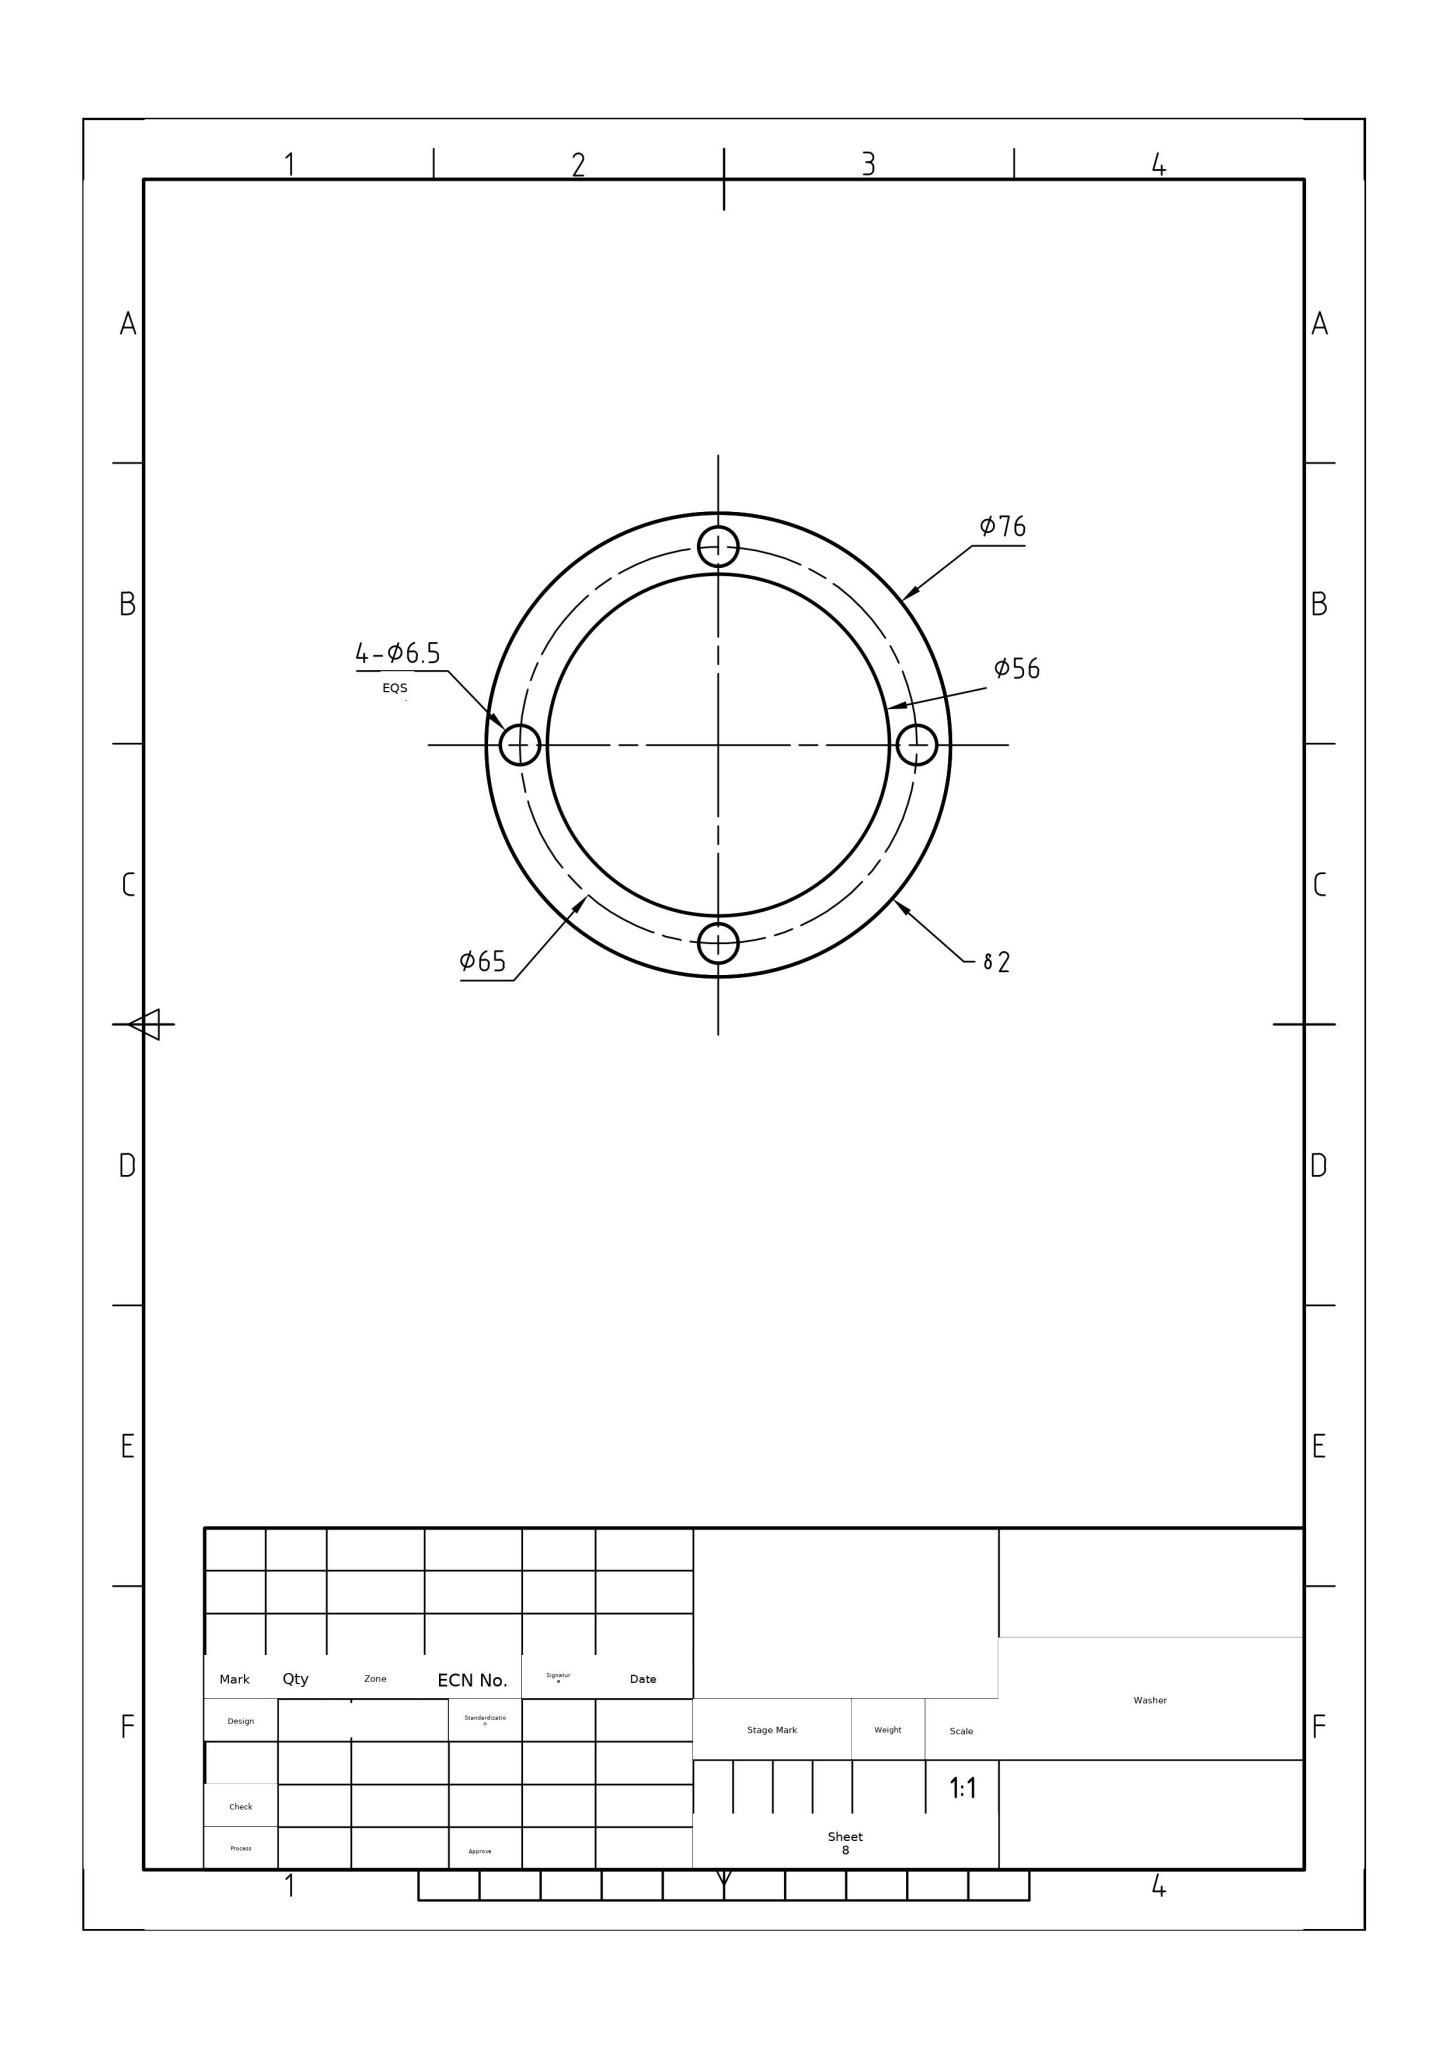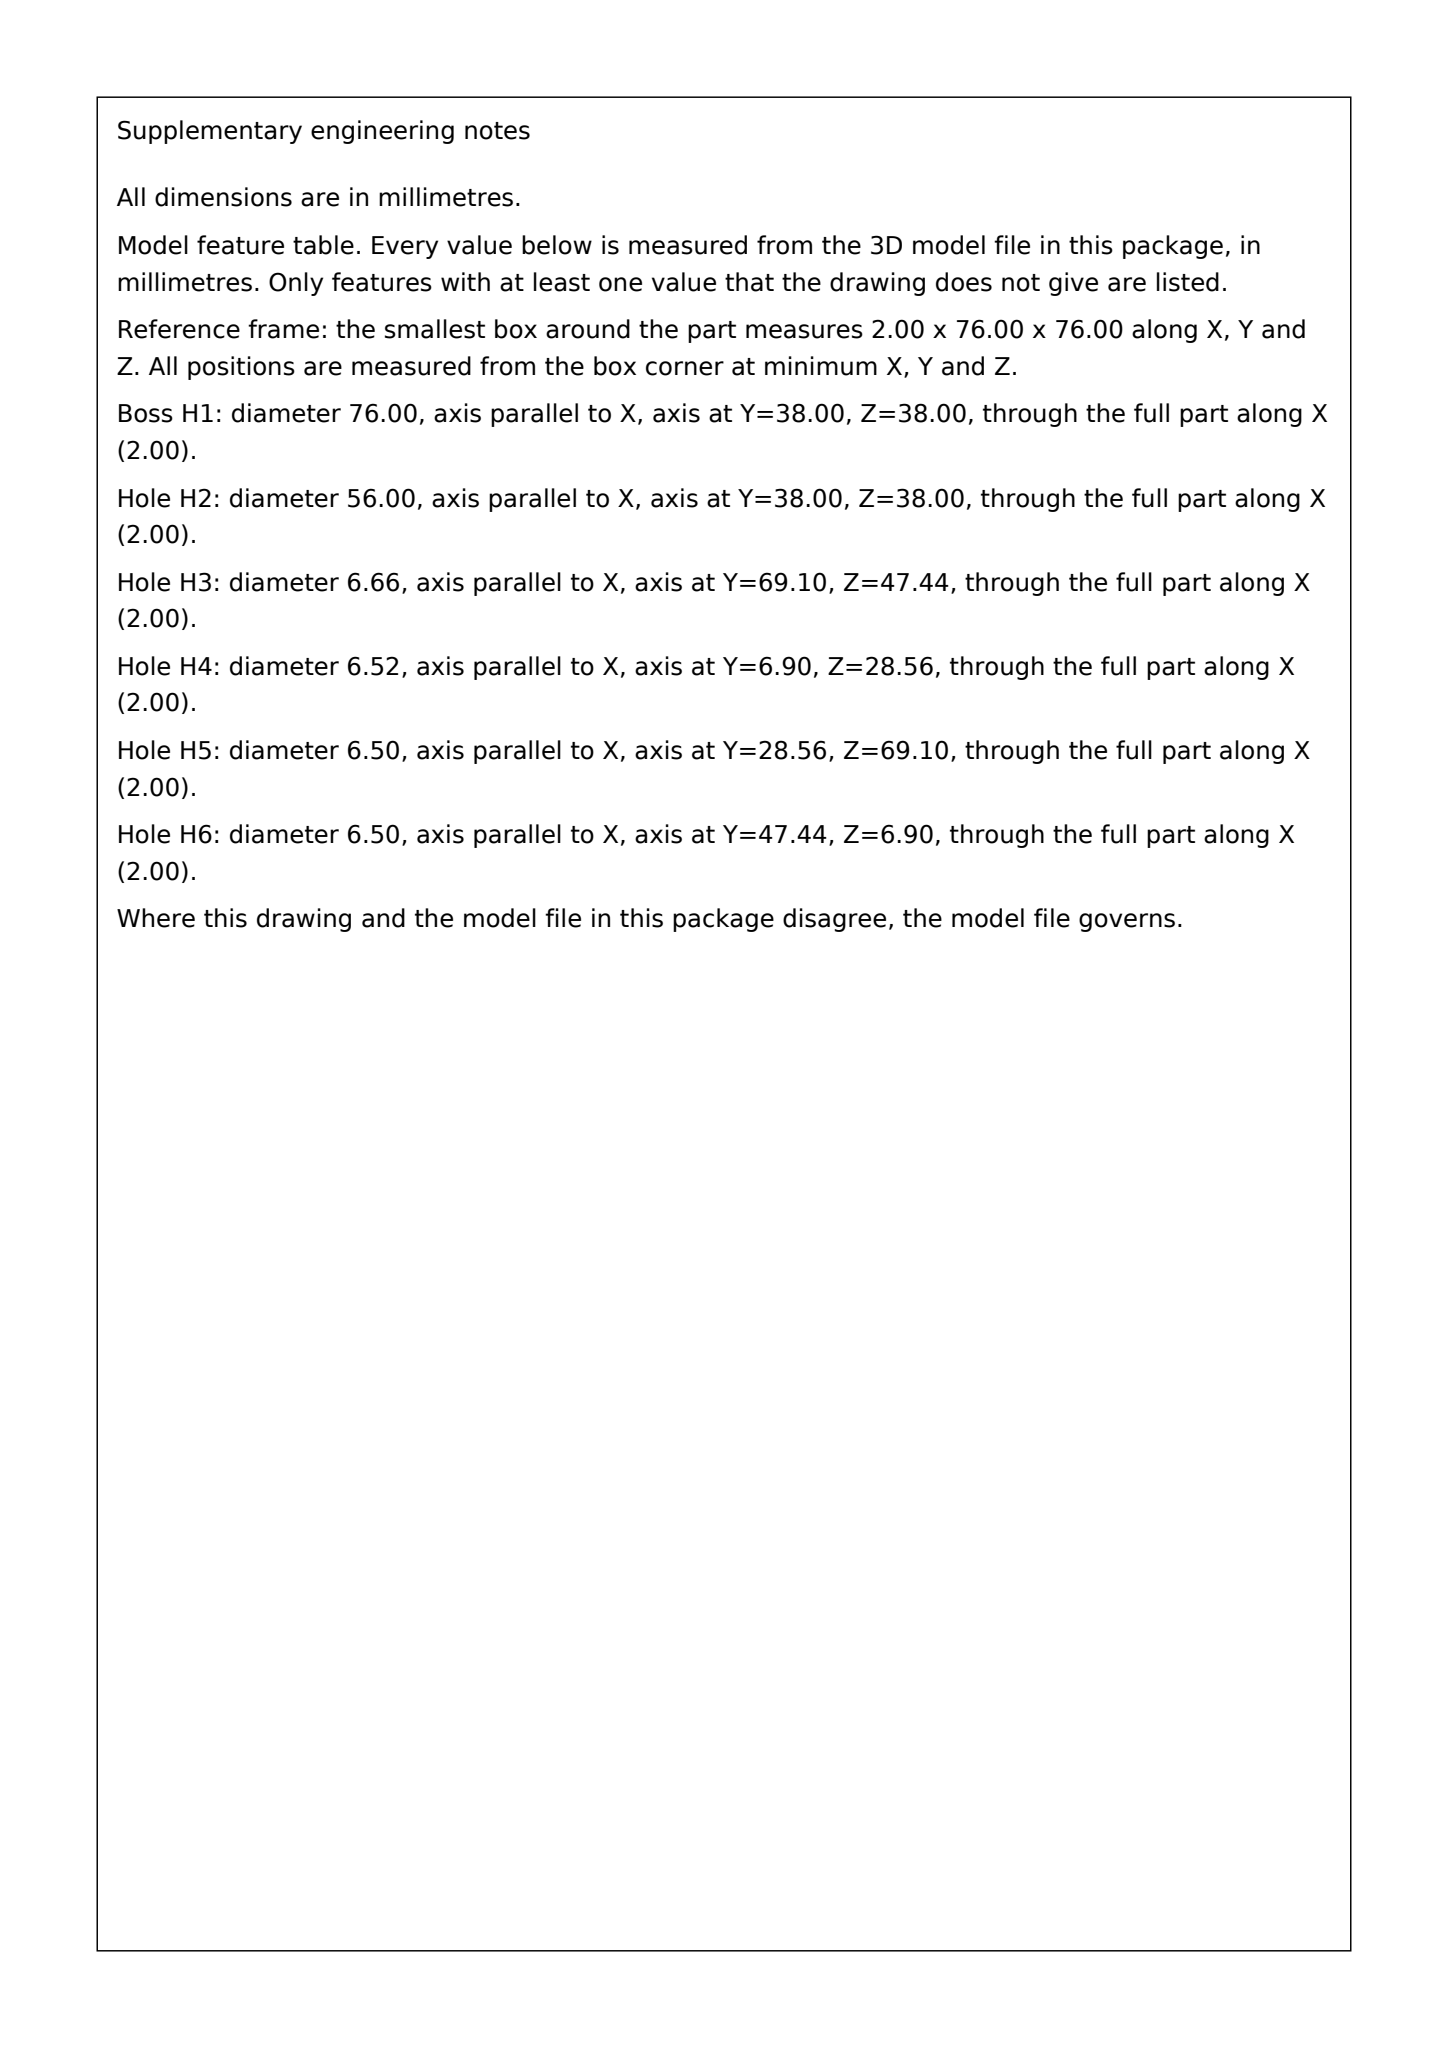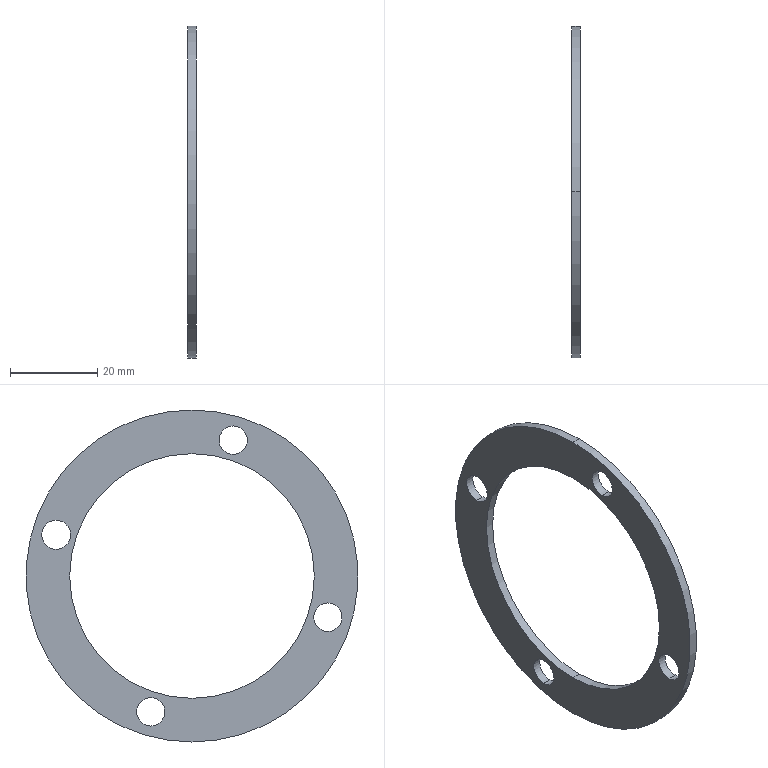Part | SolidWorks | mm | 1 solid | 14 faces | box 2 x 76 x 76 mm | volume 3878 mm3 | cylinder 12 | plane 2 | commonest cylinder face diameters 6.5 x4 6.651 x2 6.516 x2 56 x2 76 x2
build123d program:
from build123d import *

# Parameters (mm, degrees)
SKETCH2_R           = 38
SKETCH2_R_2         = 28
BOSS_EXTRUDE1_DEPTH = 2
CUT_EXTRUDE1_REACH  = 55.777
SKETCH3_R           = 3.326
SKETCH3_R_2         = 3.25
SKETCH3_R_3         = 3.258


with BuildPart() as part:
    # Sketch2 → Boss-Extrude1 (new body)
    with BuildSketch(Plane(origin=(0, 0, 0), x_dir=(0, 0, -1), z_dir=(1, 0, 0))):
        Circle(SKETCH2_R)
        Circle(SKETCH2_R_2, mode=Mode.SUBTRACT)
    extrude(amount=BOSS_EXTRUDE1_DEPTH)

    # Sketch3 → Cut-Extrude1 (cut, up to next)
    with BuildSketch(Plane.ZY, mode=Mode.PRIVATE) as cut_extrude1_sk1:
        with Locations((9.437, 31.1)):
            Circle(SKETCH3_R)
    cut_extrude1_tool1 = extrude(cut_extrude1_sk1.sketch, amount=-CUT_EXTRUDE1_REACH, mode=Mode.PRIVATE) & part.part
    # Sketch3 → Cut-Extrude1 (cut, up to next)
    with BuildSketch(Plane.ZY, mode=Mode.PRIVATE) as cut_extrude1_sk2:
        with Locations((31.1, -9.437)):
            Circle(SKETCH3_R_2)
    cut_extrude1_tool2 = extrude(cut_extrude1_sk2.sketch, amount=-CUT_EXTRUDE1_REACH, mode=Mode.PRIVATE) & part.part
    # Sketch3 → Cut-Extrude1 (cut, up to next)
    with BuildSketch(Plane.ZY, mode=Mode.PRIVATE) as cut_extrude1_sk3:
        with Locations((-9.437, -31.1)):
            Circle(SKETCH3_R_3)
    cut_extrude1_tool3 = extrude(cut_extrude1_sk3.sketch, amount=-CUT_EXTRUDE1_REACH, mode=Mode.PRIVATE) & part.part
    # Sketch3 → Cut-Extrude1 (cut, up to next)
    with BuildSketch(Plane.ZY, mode=Mode.PRIVATE) as cut_extrude1_sk4:
        with Locations((-31.1, 9.437)):
            Circle(SKETCH3_R_2)
    cut_extrude1_tool4 = extrude(cut_extrude1_sk4.sketch, amount=-CUT_EXTRUDE1_REACH, mode=Mode.PRIVATE) & part.part
    add(cut_extrude1_tool1.solids().sort_by_distance((0, 31.1, 9.437))[0], mode=Mode.SUBTRACT)
    add(cut_extrude1_tool2.solids().sort_by_distance((0, -9.437, 31.1))[0], mode=Mode.SUBTRACT)
    add(cut_extrude1_tool3.solids().sort_by_distance((0, -31.1, -9.437))[0], mode=Mode.SUBTRACT)
    add(cut_extrude1_tool4.solids().sort_by_distance((0, 9.437, -31.1))[0], mode=Mode.SUBTRACT)


solid = part.part
STEP:
#1=CARTESIAN_POINT('',(2.,31.1,6.111));
#2=VERTEX_POINT('',#1);
#3=CARTESIAN_POINT('',(2.,31.1,12.763));
#4=VERTEX_POINT('',#3);
#5=CARTESIAN_POINT('',(2.,31.1,9.437));
#6=DIRECTION('',(-1.,0.,0.));
#7=DIRECTION('',(0.,0.,-1.));
#8=AXIS2_PLACEMENT_3D('',#5,#6,#7);
#9=CIRCLE('',#8,3.326);
#10=EDGE_CURVE('',#2,#4,#9,.T.);
#11=ORIENTED_EDGE('',*,*,#10,.F.);
#12=CARTESIAN_POINT('',(0.,31.1,6.111));
#13=VERTEX_POINT('',#12);
#14=CARTESIAN_POINT('',(2.001,31.1,6.111));
#15=DIRECTION('',(-1.,0.,0.));
#16=VECTOR('',#15,1000.);
#17=LINE('',#14,#16);
#18=EDGE_CURVE('',#2,#13,#17,.T.);
#19=ORIENTED_EDGE('',*,*,#18,.T.);
#20=CARTESIAN_POINT('',(0.,31.1,12.763));
#21=VERTEX_POINT('',#20);
#22=CARTESIAN_POINT('',(0.,31.1,9.437));
#23=DIRECTION('',(-1.,0.,0.));
#24=DIRECTION('',(0.,0.,1.));
#25=AXIS2_PLACEMENT_3D('',#22,#23,#24);
#26=CIRCLE('',#25,3.326);
#27=EDGE_CURVE('',#13,#21,#26,.T.);
#28=ORIENTED_EDGE('',*,*,#27,.T.);
#29=CARTESIAN_POINT('',(2.001,31.1,12.763));
#30=DIRECTION('',(-1.,0.,0.));
#31=VECTOR('',#30,1000.);
#32=LINE('',#29,#31);
#33=EDGE_CURVE('',#4,#21,#32,.T.);
#34=ORIENTED_EDGE('',*,*,#33,.F.);
#35=EDGE_LOOP('',(#11,#19,#28,#34));
#36=FACE_OUTER_BOUND('',#35,.T.);
#37=CARTESIAN_POINT('',(2.001,31.1,9.437));
#38=DIRECTION('',(-1.,0.,0.));
#39=DIRECTION('',(0.,0.,1.));
#40=AXIS2_PLACEMENT_3D('',#37,#38,#39);
#41=CYLINDRICAL_SURFACE('',#40,3.326);
#42=ADVANCED_FACE('',(#36),#41,.F.);
#43=CARTESIAN_POINT('',(2.,-9.437,27.85));
#44=VERTEX_POINT('',#43);
#45=CARTESIAN_POINT('',(2.,-9.437,34.35));
#46=VERTEX_POINT('',#45);
#47=CARTESIAN_POINT('',(2.,-9.437,31.1));
#48=DIRECTION('',(-1.,0.,0.));
#49=DIRECTION('',(0.,0.,-1.));
#50=AXIS2_PLACEMENT_3D('',#47,#48,#49);
#51=CIRCLE('',#50,3.25);
#52=EDGE_CURVE('',#44,#46,#51,.T.);
#53=ORIENTED_EDGE('',*,*,#52,.F.);
#54=CARTESIAN_POINT('',(0.,-9.437,27.85));
#55=VERTEX_POINT('',#54);
#56=CARTESIAN_POINT('',(2.001,-9.437,27.85));
#57=DIRECTION('',(-1.,0.,0.));
#58=VECTOR('',#57,1000.);
#59=LINE('',#56,#58);
#60=EDGE_CURVE('',#44,#55,#59,.T.);
#61=ORIENTED_EDGE('',*,*,#60,.T.);
#62=CARTESIAN_POINT('',(0.,-9.437,34.35));
#63=VERTEX_POINT('',#62);
#64=CARTESIAN_POINT('',(0.,-9.437,31.1));
#65=DIRECTION('',(-1.,0.,0.));
#66=DIRECTION('',(0.,0.,1.));
#67=AXIS2_PLACEMENT_3D('',#64,#65,#66);
#68=CIRCLE('',#67,3.25);
#69=EDGE_CURVE('',#55,#63,#68,.T.);
#70=ORIENTED_EDGE('',*,*,#69,.T.);
#71=CARTESIAN_POINT('',(2.001,-9.437,34.35));
#72=DIRECTION('',(-1.,0.,0.));
#73=VECTOR('',#72,1000.);
#74=LINE('',#71,#73);
#75=EDGE_CURVE('',#46,#63,#74,.T.);
#76=ORIENTED_EDGE('',*,*,#75,.F.);
#77=EDGE_LOOP('',(#53,#61,#70,#76));
#78=FACE_OUTER_BOUND('',#77,.T.);
#79=CARTESIAN_POINT('',(2.001,-9.437,31.1));
#80=DIRECTION('',(-1.,0.,0.));
#81=DIRECTION('',(0.,0.,1.));
#82=AXIS2_PLACEMENT_3D('',#79,#80,#81);
#83=CYLINDRICAL_SURFACE('',#82,3.25);
#84=ADVANCED_FACE('',(#78),#83,.F.);
#85=CARTESIAN_POINT('',(2.,-31.1,-12.695));
#86=VERTEX_POINT('',#85);
#87=CARTESIAN_POINT('',(2.,-31.1,-6.179));
#88=VERTEX_POINT('',#87);
#89=CARTESIAN_POINT('',(2.,-31.1,-9.437));
#90=DIRECTION('',(-1.,0.,0.));
#91=DIRECTION('',(0.,0.,-1.));
#92=AXIS2_PLACEMENT_3D('',#89,#90,#91);
#93=CIRCLE('',#92,3.258);
#94=EDGE_CURVE('',#86,#88,#93,.T.);
#95=ORIENTED_EDGE('',*,*,#94,.F.);
#96=CARTESIAN_POINT('',(0.,-31.1,-12.695));
#97=VERTEX_POINT('',#96);
#98=CARTESIAN_POINT('',(2.001,-31.1,-12.695));
#99=DIRECTION('',(-1.,0.,0.));
#100=VECTOR('',#99,1000.);
#101=LINE('',#98,#100);
#102=EDGE_CURVE('',#86,#97,#101,.T.);
#103=ORIENTED_EDGE('',*,*,#102,.T.);
#104=CARTESIAN_POINT('',(0.,-31.1,-6.179));
#105=VERTEX_POINT('',#104);
#106=CARTESIAN_POINT('',(0.,-31.1,-9.437));
#107=DIRECTION('',(-1.,0.,0.));
#108=DIRECTION('',(0.,0.,1.));
#109=AXIS2_PLACEMENT_3D('',#106,#107,#108);
#110=CIRCLE('',#109,3.258);
#111=EDGE_CURVE('',#97,#105,#110,.T.);
#112=ORIENTED_EDGE('',*,*,#111,.T.);
#113=CARTESIAN_POINT('',(2.001,-31.1,-6.179));
#114=DIRECTION('',(-1.,0.,0.));
#115=VECTOR('',#114,1000.);
#116=LINE('',#113,#115);
#117=EDGE_CURVE('',#88,#105,#116,.T.);
#118=ORIENTED_EDGE('',*,*,#117,.F.);
#119=EDGE_LOOP('',(#95,#103,#112,#118));
#120=FACE_OUTER_BOUND('',#119,.T.);
#121=CARTESIAN_POINT('',(2.001,-31.1,-9.437));
#122=DIRECTION('',(-1.,0.,0.));
#123=DIRECTION('',(0.,0.,1.));
#124=AXIS2_PLACEMENT_3D('',#121,#122,#123);
#125=CYLINDRICAL_SURFACE('',#124,3.258);
#126=ADVANCED_FACE('',(#120),#125,.F.);
#127=CARTESIAN_POINT('',(2.,9.437,-34.35));
#128=VERTEX_POINT('',#127);
#129=CARTESIAN_POINT('',(2.,9.437,-27.85));
#130=VERTEX_POINT('',#129);
#131=CARTESIAN_POINT('',(2.,9.437,-31.1));
#132=DIRECTION('',(-1.,0.,0.));
#133=DIRECTION('',(0.,0.,-1.));
#134=AXIS2_PLACEMENT_3D('',#131,#132,#133);
#135=CIRCLE('',#134,3.25);
#136=EDGE_CURVE('',#128,#130,#135,.T.);
#137=ORIENTED_EDGE('',*,*,#136,.F.);
#138=CARTESIAN_POINT('',(0.,9.437,-34.35));
#139=VERTEX_POINT('',#138);
#140=CARTESIAN_POINT('',(2.001,9.437,-34.35));
#141=DIRECTION('',(-1.,0.,0.));
#142=VECTOR('',#141,1000.);
#143=LINE('',#140,#142);
#144=EDGE_CURVE('',#128,#139,#143,.T.);
#145=ORIENTED_EDGE('',*,*,#144,.T.);
#146=CARTESIAN_POINT('',(0.,9.437,-27.85));
#147=VERTEX_POINT('',#146);
#148=CARTESIAN_POINT('',(0.,9.437,-31.1));
#149=DIRECTION('',(-1.,0.,0.));
#150=DIRECTION('',(0.,0.,1.));
#151=AXIS2_PLACEMENT_3D('',#148,#149,#150);
#152=CIRCLE('',#151,3.25);
#153=EDGE_CURVE('',#139,#147,#152,.T.);
#154=ORIENTED_EDGE('',*,*,#153,.T.);
#155=CARTESIAN_POINT('',(2.001,9.437,-27.85));
#156=DIRECTION('',(-1.,0.,0.));
#157=VECTOR('',#156,1000.);
#158=LINE('',#155,#157);
#159=EDGE_CURVE('',#130,#147,#158,.T.);
#160=ORIENTED_EDGE('',*,*,#159,.F.);
#161=EDGE_LOOP('',(#137,#145,#154,#160));
#162=FACE_OUTER_BOUND('',#161,.T.);
#163=CARTESIAN_POINT('',(2.001,9.437,-31.1));
#164=DIRECTION('',(-1.,0.,0.));
#165=DIRECTION('',(0.,0.,1.));
#166=AXIS2_PLACEMENT_3D('',#163,#164,#165);
#167=CYLINDRICAL_SURFACE('',#166,3.25);
#168=ADVANCED_FACE('',(#162),#167,.F.);
#169=CARTESIAN_POINT('',(2.,0.,28.));
#170=VERTEX_POINT('',#169);
#171=CARTESIAN_POINT('',(2.,0.,-28.));
#172=VERTEX_POINT('',#171);
#173=CARTESIAN_POINT('',(2.,0.,0.));
#174=DIRECTION('',(1.,0.,0.));
#175=DIRECTION('',(0.,0.,-1.));
#176=AXIS2_PLACEMENT_3D('',#173,#174,#175);
#177=CIRCLE('',#176,28.);
#178=EDGE_CURVE('',#170,#172,#177,.T.);
#179=ORIENTED_EDGE('',*,*,#178,.T.);
#180=CARTESIAN_POINT('',(0.,0.,-28.));
#181=VERTEX_POINT('',#180);
#182=CARTESIAN_POINT('',(2.,0.,-28.));
#183=DIRECTION('',(-1.,0.,0.));
#184=VECTOR('',#183,1000.);
#185=LINE('',#182,#184);
#186=EDGE_CURVE('',#172,#181,#185,.T.);
#187=ORIENTED_EDGE('',*,*,#186,.T.);
#188=CARTESIAN_POINT('',(0.,0.,28.));
#189=VERTEX_POINT('',#188);
#190=CARTESIAN_POINT('',(0.,0.,0.));
#191=DIRECTION('',(1.,0.,0.));
#192=DIRECTION('',(0.,0.,-1.));
#193=AXIS2_PLACEMENT_3D('',#190,#191,#192);
#194=CIRCLE('',#193,28.);
#195=EDGE_CURVE('',#189,#181,#194,.T.);
#196=ORIENTED_EDGE('',*,*,#195,.F.);
#197=CARTESIAN_POINT('',(2.,0.,28.));
#198=DIRECTION('',(-1.,0.,0.));
#199=VECTOR('',#198,1000.);
#200=LINE('',#197,#199);
#201=EDGE_CURVE('',#170,#189,#200,.T.);
#202=ORIENTED_EDGE('',*,*,#201,.F.);
#203=EDGE_LOOP('',(#179,#187,#196,#202));
#204=FACE_OUTER_BOUND('',#203,.T.);
#205=CARTESIAN_POINT('',(2.,0.,0.));
#206=DIRECTION('',(-1.,0.,0.));
#207=DIRECTION('',(0.,0.,1.));
#208=AXIS2_PLACEMENT_3D('',#205,#206,#207);
#209=CYLINDRICAL_SURFACE('',#208,28.);
#210=ADVANCED_FACE('',(#204),#209,.F.);
#211=CARTESIAN_POINT('',(2.,0.,-38.));
#212=VERTEX_POINT('',#211);
#213=CARTESIAN_POINT('',(2.,0.,38.));
#214=VERTEX_POINT('',#213);
#215=CARTESIAN_POINT('',(2.,0.,0.));
#216=DIRECTION('',(1.,0.,0.));
#217=DIRECTION('',(0.,0.,-1.));
#218=AXIS2_PLACEMENT_3D('',#215,#216,#217);
#219=CIRCLE('',#218,38.);
#220=EDGE_CURVE('',#212,#214,#219,.T.);
#221=ORIENTED_EDGE('',*,*,#220,.F.);
#222=CARTESIAN_POINT('',(0.,0.,-38.));
#223=VERTEX_POINT('',#222);
#224=CARTESIAN_POINT('',(2.,0.,-38.));
#225=DIRECTION('',(-1.,0.,0.));
#226=VECTOR('',#225,1000.);
#227=LINE('',#224,#226);
#228=EDGE_CURVE('',#212,#223,#227,.T.);
#229=ORIENTED_EDGE('',*,*,#228,.T.);
#230=CARTESIAN_POINT('',(0.,0.,38.));
#231=VERTEX_POINT('',#230);
#232=CARTESIAN_POINT('',(0.,0.,0.));
#233=DIRECTION('',(1.,0.,0.));
#234=DIRECTION('',(0.,0.,-1.));
#235=AXIS2_PLACEMENT_3D('',#232,#233,#234);
#236=CIRCLE('',#235,38.);
#237=EDGE_CURVE('',#223,#231,#236,.T.);
#238=ORIENTED_EDGE('',*,*,#237,.T.);
#239=CARTESIAN_POINT('',(2.,0.,38.));
#240=DIRECTION('',(-1.,0.,0.));
#241=VECTOR('',#240,1000.);
#242=LINE('',#239,#241);
#243=EDGE_CURVE('',#214,#231,#242,.T.);
#244=ORIENTED_EDGE('',*,*,#243,.F.);
#245=EDGE_LOOP('',(#221,#229,#238,#244));
#246=FACE_OUTER_BOUND('',#245,.T.);
#247=CARTESIAN_POINT('',(2.,0.,0.));
#248=DIRECTION('',(-1.,0.,0.));
#249=DIRECTION('',(0.,0.,1.));
#250=AXIS2_PLACEMENT_3D('',#247,#248,#249);
#251=CYLINDRICAL_SURFACE('',#250,38.);
#252=ADVANCED_FACE('',(#246),#251,.T.);
#253=CARTESIAN_POINT('',(2.,31.1,9.437));
#254=DIRECTION('',(-1.,0.,0.));
#255=DIRECTION('',(0.,0.,-1.));
#256=AXIS2_PLACEMENT_3D('',#253,#254,#255);
#257=CIRCLE('',#256,3.326);
#258=EDGE_CURVE('',#4,#2,#257,.T.);
#259=ORIENTED_EDGE('',*,*,#258,.T.);
#260=ORIENTED_EDGE('',*,*,#10,.T.);
#261=EDGE_LOOP('',(#259,#260));
#262=FACE_BOUND('',#261,.T.);
#263=CARTESIAN_POINT('',(2.,-9.437,31.1));
#264=DIRECTION('',(-1.,0.,0.));
#265=DIRECTION('',(0.,0.,-1.));
#266=AXIS2_PLACEMENT_3D('',#263,#264,#265);
#267=CIRCLE('',#266,3.25);
#268=EDGE_CURVE('',#46,#44,#267,.T.);
#269=ORIENTED_EDGE('',*,*,#268,.T.);
#270=ORIENTED_EDGE('',*,*,#52,.T.);
#271=EDGE_LOOP('',(#269,#270));
#272=FACE_BOUND('',#271,.T.);
#273=CARTESIAN_POINT('',(2.,-31.1,-9.437));
#274=DIRECTION('',(-1.,0.,0.));
#275=DIRECTION('',(0.,0.,-1.));
#276=AXIS2_PLACEMENT_3D('',#273,#274,#275);
#277=CIRCLE('',#276,3.258);
#278=EDGE_CURVE('',#88,#86,#277,.T.);
#279=ORIENTED_EDGE('',*,*,#278,.T.);
#280=ORIENTED_EDGE('',*,*,#94,.T.);
#281=EDGE_LOOP('',(#279,#280));
#282=FACE_BOUND('',#281,.T.);
#283=CARTESIAN_POINT('',(2.,9.437,-31.1));
#284=DIRECTION('',(-1.,0.,0.));
#285=DIRECTION('',(0.,0.,-1.));
#286=AXIS2_PLACEMENT_3D('',#283,#284,#285);
#287=CIRCLE('',#286,3.25);
#288=EDGE_CURVE('',#130,#128,#287,.T.);
#289=ORIENTED_EDGE('',*,*,#288,.T.);
#290=ORIENTED_EDGE('',*,*,#136,.T.);
#291=EDGE_LOOP('',(#289,#290));
#292=FACE_BOUND('',#291,.T.);
#293=CARTESIAN_POINT('',(2.,0.,0.));
#294=DIRECTION('',(1.,0.,0.));
#295=DIRECTION('',(0.,0.,-1.));
#296=AXIS2_PLACEMENT_3D('',#293,#294,#295);
#297=CIRCLE('',#296,38.);
#298=EDGE_CURVE('',#214,#212,#297,.T.);
#299=ORIENTED_EDGE('',*,*,#298,.T.);
#300=ORIENTED_EDGE('',*,*,#220,.T.);
#301=EDGE_LOOP('',(#299,#300));
#302=FACE_OUTER_BOUND('',#301,.T.);
#303=ORIENTED_EDGE('',*,*,#178,.F.);
#304=CARTESIAN_POINT('',(2.,0.,0.));
#305=DIRECTION('',(1.,0.,0.));
#306=DIRECTION('',(0.,0.,-1.));
#307=AXIS2_PLACEMENT_3D('',#304,#305,#306);
#308=CIRCLE('',#307,28.);
#309=EDGE_CURVE('',#172,#170,#308,.T.);
#310=ORIENTED_EDGE('',*,*,#309,.F.);
#311=EDGE_LOOP('',(#303,#310));
#312=FACE_BOUND('',#311,.T.);
#313=CARTESIAN_POINT('',(2.,0.,0.));
#314=DIRECTION('',(1.,0.,0.));
#315=DIRECTION('',(0.,0.,-1.));
#316=AXIS2_PLACEMENT_3D('',#313,#314,#315);
#317=PLANE('',#316);
#318=ADVANCED_FACE('',(#262,#272,#282,#292,#302,#312),#317,.T.);
#319=CARTESIAN_POINT('',(0.,31.1,9.437));
#320=DIRECTION('',(-1.,0.,0.));
#321=DIRECTION('',(0.,0.,1.));
#322=AXIS2_PLACEMENT_3D('',#319,#320,#321);
#323=CIRCLE('',#322,3.326);
#324=EDGE_CURVE('',#21,#13,#323,.T.);
#325=ORIENTED_EDGE('',*,*,#324,.F.);
#326=ORIENTED_EDGE('',*,*,#27,.F.);
#327=EDGE_LOOP('',(#325,#326));
#328=FACE_BOUND('',#327,.T.);
#329=CARTESIAN_POINT('',(0.,-9.437,31.1));
#330=DIRECTION('',(-1.,0.,0.));
#331=DIRECTION('',(0.,0.,1.));
#332=AXIS2_PLACEMENT_3D('',#329,#330,#331);
#333=CIRCLE('',#332,3.25);
#334=EDGE_CURVE('',#63,#55,#333,.T.);
#335=ORIENTED_EDGE('',*,*,#334,.F.);
#336=ORIENTED_EDGE('',*,*,#69,.F.);
#337=EDGE_LOOP('',(#335,#336));
#338=FACE_BOUND('',#337,.T.);
#339=CARTESIAN_POINT('',(0.,-31.1,-9.437));
#340=DIRECTION('',(-1.,0.,0.));
#341=DIRECTION('',(0.,0.,1.));
#342=AXIS2_PLACEMENT_3D('',#339,#340,#341);
#343=CIRCLE('',#342,3.258);
#344=EDGE_CURVE('',#105,#97,#343,.T.);
#345=ORIENTED_EDGE('',*,*,#344,.F.);
#346=ORIENTED_EDGE('',*,*,#111,.F.);
#347=EDGE_LOOP('',(#345,#346));
#348=FACE_BOUND('',#347,.T.);
#349=CARTESIAN_POINT('',(0.,9.437,-31.1));
#350=DIRECTION('',(-1.,0.,0.));
#351=DIRECTION('',(0.,0.,1.));
#352=AXIS2_PLACEMENT_3D('',#349,#350,#351);
#353=CIRCLE('',#352,3.25);
#354=EDGE_CURVE('',#147,#139,#353,.T.);
#355=ORIENTED_EDGE('',*,*,#354,.F.);
#356=ORIENTED_EDGE('',*,*,#153,.F.);
#357=EDGE_LOOP('',(#355,#356));
#358=FACE_BOUND('',#357,.T.);
#359=CARTESIAN_POINT('',(0.,0.,0.));
#360=DIRECTION('',(1.,0.,0.));
#361=DIRECTION('',(0.,0.,-1.));
#362=AXIS2_PLACEMENT_3D('',#359,#360,#361);
#363=CIRCLE('',#362,38.);
#364=EDGE_CURVE('',#231,#223,#363,.T.);
#365=ORIENTED_EDGE('',*,*,#364,.F.);
#366=ORIENTED_EDGE('',*,*,#237,.F.);
#367=EDGE_LOOP('',(#365,#366));
#368=FACE_OUTER_BOUND('',#367,.T.);
#369=ORIENTED_EDGE('',*,*,#195,.T.);
#370=CARTESIAN_POINT('',(0.,0.,0.));
#371=DIRECTION('',(1.,0.,0.));
#372=DIRECTION('',(0.,0.,-1.));
#373=AXIS2_PLACEMENT_3D('',#370,#371,#372);
#374=CIRCLE('',#373,28.);
#375=EDGE_CURVE('',#181,#189,#374,.T.);
#376=ORIENTED_EDGE('',*,*,#375,.T.);
#377=EDGE_LOOP('',(#369,#376));
#378=FACE_BOUND('',#377,.T.);
#379=CARTESIAN_POINT('',(0.,0.,0.));
#380=DIRECTION('',(1.,0.,0.));
#381=DIRECTION('',(0.,0.,-1.));
#382=AXIS2_PLACEMENT_3D('',#379,#380,#381);
#383=PLANE('',#382);
#384=ADVANCED_FACE('',(#328,#338,#348,#358,#368,#378),#383,.F.);
#385=ORIENTED_EDGE('',*,*,#228,.F.);
#386=ORIENTED_EDGE('',*,*,#298,.F.);
#387=ORIENTED_EDGE('',*,*,#243,.T.);
#388=ORIENTED_EDGE('',*,*,#364,.T.);
#389=EDGE_LOOP('',(#385,#386,#387,#388));
#390=FACE_OUTER_BOUND('',#389,.T.);
#391=CARTESIAN_POINT('',(2.,0.,0.));
#392=DIRECTION('',(-1.,0.,0.));
#393=DIRECTION('',(0.,0.,1.));
#394=AXIS2_PLACEMENT_3D('',#391,#392,#393);
#395=CYLINDRICAL_SURFACE('',#394,38.);
#396=ADVANCED_FACE('',(#390),#395,.T.);
#397=ORIENTED_EDGE('',*,*,#186,.F.);
#398=ORIENTED_EDGE('',*,*,#309,.T.);
#399=ORIENTED_EDGE('',*,*,#201,.T.);
#400=ORIENTED_EDGE('',*,*,#375,.F.);
#401=EDGE_LOOP('',(#397,#398,#399,#400));
#402=FACE_OUTER_BOUND('',#401,.T.);
#403=CARTESIAN_POINT('',(2.,0.,0.));
#404=DIRECTION('',(-1.,0.,0.));
#405=DIRECTION('',(0.,0.,1.));
#406=AXIS2_PLACEMENT_3D('',#403,#404,#405);
#407=CYLINDRICAL_SURFACE('',#406,28.);
#408=ADVANCED_FACE('',(#402),#407,.F.);
#409=ORIENTED_EDGE('',*,*,#144,.F.);
#410=ORIENTED_EDGE('',*,*,#288,.F.);
#411=ORIENTED_EDGE('',*,*,#159,.T.);
#412=ORIENTED_EDGE('',*,*,#354,.T.);
#413=EDGE_LOOP('',(#409,#410,#411,#412));
#414=FACE_OUTER_BOUND('',#413,.T.);
#415=CARTESIAN_POINT('',(2.001,9.437,-31.1));
#416=DIRECTION('',(-1.,0.,0.));
#417=DIRECTION('',(0.,0.,1.));
#418=AXIS2_PLACEMENT_3D('',#415,#416,#417);
#419=CYLINDRICAL_SURFACE('',#418,3.25);
#420=ADVANCED_FACE('',(#414),#419,.F.);
#421=ORIENTED_EDGE('',*,*,#102,.F.);
#422=ORIENTED_EDGE('',*,*,#278,.F.);
#423=ORIENTED_EDGE('',*,*,#117,.T.);
#424=ORIENTED_EDGE('',*,*,#344,.T.);
#425=EDGE_LOOP('',(#421,#422,#423,#424));
#426=FACE_OUTER_BOUND('',#425,.T.);
#427=CARTESIAN_POINT('',(2.001,-31.1,-9.437));
#428=DIRECTION('',(-1.,0.,0.));
#429=DIRECTION('',(0.,0.,1.));
#430=AXIS2_PLACEMENT_3D('',#427,#428,#429);
#431=CYLINDRICAL_SURFACE('',#430,3.258);
#432=ADVANCED_FACE('',(#426),#431,.F.);
#433=ORIENTED_EDGE('',*,*,#60,.F.);
#434=ORIENTED_EDGE('',*,*,#268,.F.);
#435=ORIENTED_EDGE('',*,*,#75,.T.);
#436=ORIENTED_EDGE('',*,*,#334,.T.);
#437=EDGE_LOOP('',(#433,#434,#435,#436));
#438=FACE_OUTER_BOUND('',#437,.T.);
#439=CARTESIAN_POINT('',(2.001,-9.437,31.1));
#440=DIRECTION('',(-1.,0.,0.));
#441=DIRECTION('',(0.,0.,1.));
#442=AXIS2_PLACEMENT_3D('',#439,#440,#441);
#443=CYLINDRICAL_SURFACE('',#442,3.25);
#444=ADVANCED_FACE('',(#438),#443,.F.);
#445=ORIENTED_EDGE('',*,*,#18,.F.);
#446=ORIENTED_EDGE('',*,*,#258,.F.);
#447=ORIENTED_EDGE('',*,*,#33,.T.);
#448=ORIENTED_EDGE('',*,*,#324,.T.);
#449=EDGE_LOOP('',(#445,#446,#447,#448));
#450=FACE_OUTER_BOUND('',#449,.T.);
#451=CARTESIAN_POINT('',(2.001,31.1,9.437));
#452=DIRECTION('',(-1.,0.,0.));
#453=DIRECTION('',(0.,0.,1.));
#454=AXIS2_PLACEMENT_3D('',#451,#452,#453);
#455=CYLINDRICAL_SURFACE('',#454,3.326);
#456=ADVANCED_FACE('',(#450),#455,.F.);
#457=CLOSED_SHELL('',(#42,#84,#126,#168,#210,#252,#318,#384,#396,#408,#420,#432,#444,#456));
#458=MANIFOLD_SOLID_BREP('',#457);
#459=CARTESIAN_POINT('',(0.,0.,0.));
#460=DIRECTION('',(0.,0.,1.));
#461=DIRECTION('',(1.,0.,0.));
#462=AXIS2_PLACEMENT_3D('',#459,#460,#461);
#463=(LENGTH_UNIT()NAMED_UNIT(*)SI_UNIT(.MILLI.,.METRE.));
#464=UNCERTAINTY_MEASURE_WITH_UNIT(LENGTH_MEASURE(0.00001),#463,'','');
#465=(NAMED_UNIT(*)PLANE_ANGLE_UNIT()SI_UNIT($,.RADIAN.));
#466=(NAMED_UNIT(*)SI_UNIT($,.STERADIAN.)SOLID_ANGLE_UNIT());
#467=(GEOMETRIC_REPRESENTATION_CONTEXT(3)GLOBAL_UNCERTAINTY_ASSIGNED_CONTEXT((#464))GLOBAL_UNIT_ASSIGNED_CONTEXT((#463,#465,#466))REPRESENTATION_CONTEXT('',''));
#468=ADVANCED_BREP_SHAPE_REPRESENTATION('',(#458,#462),#467);